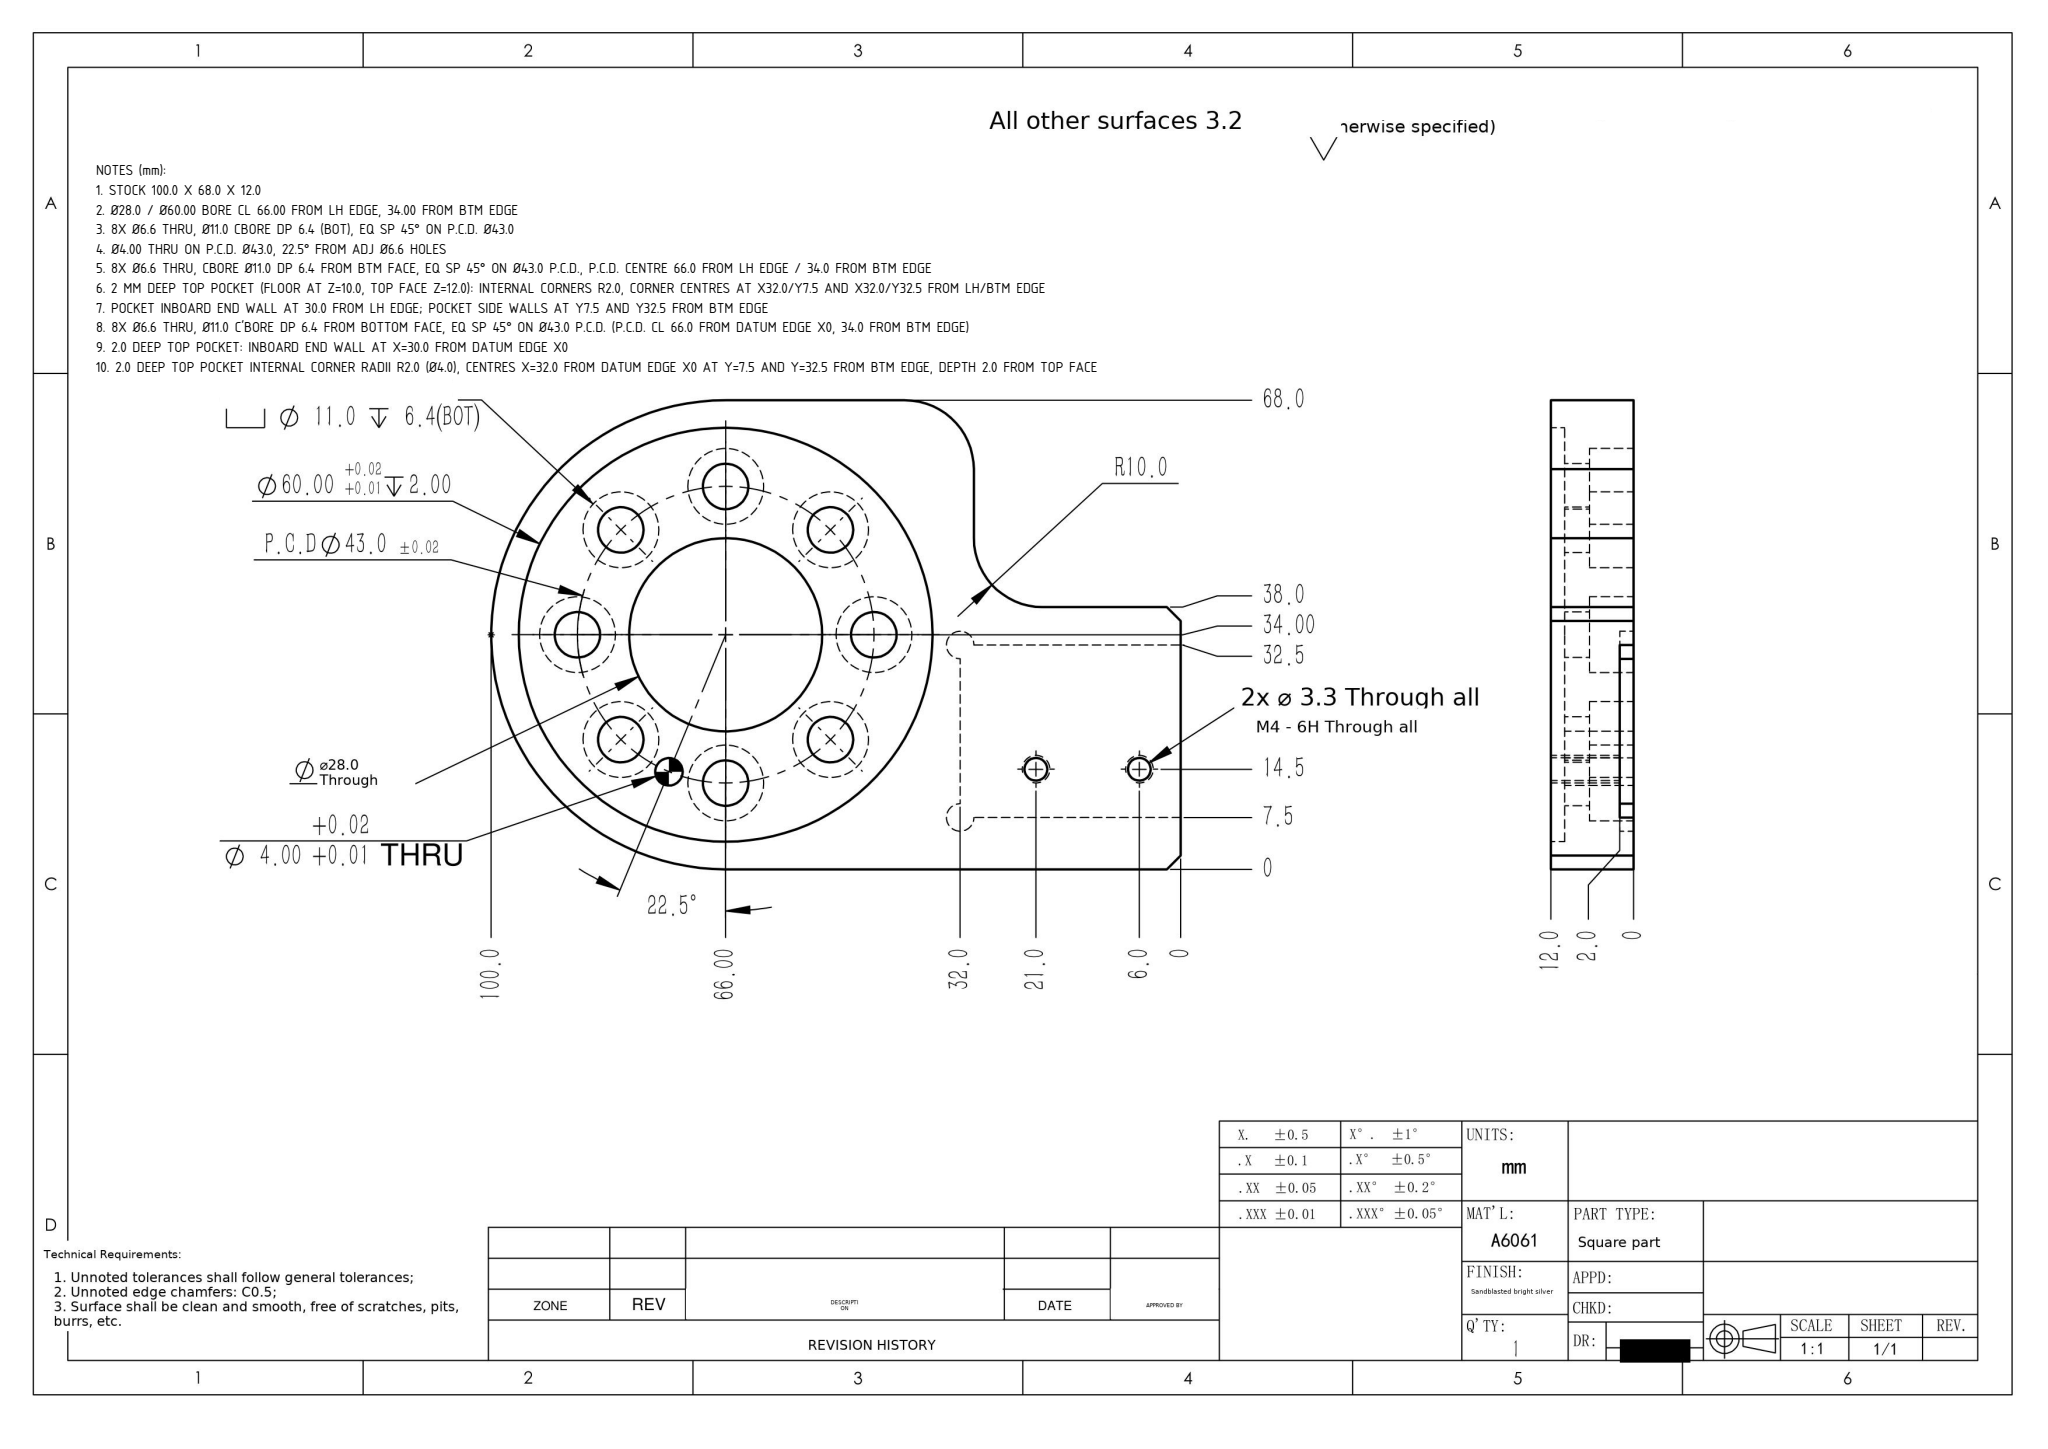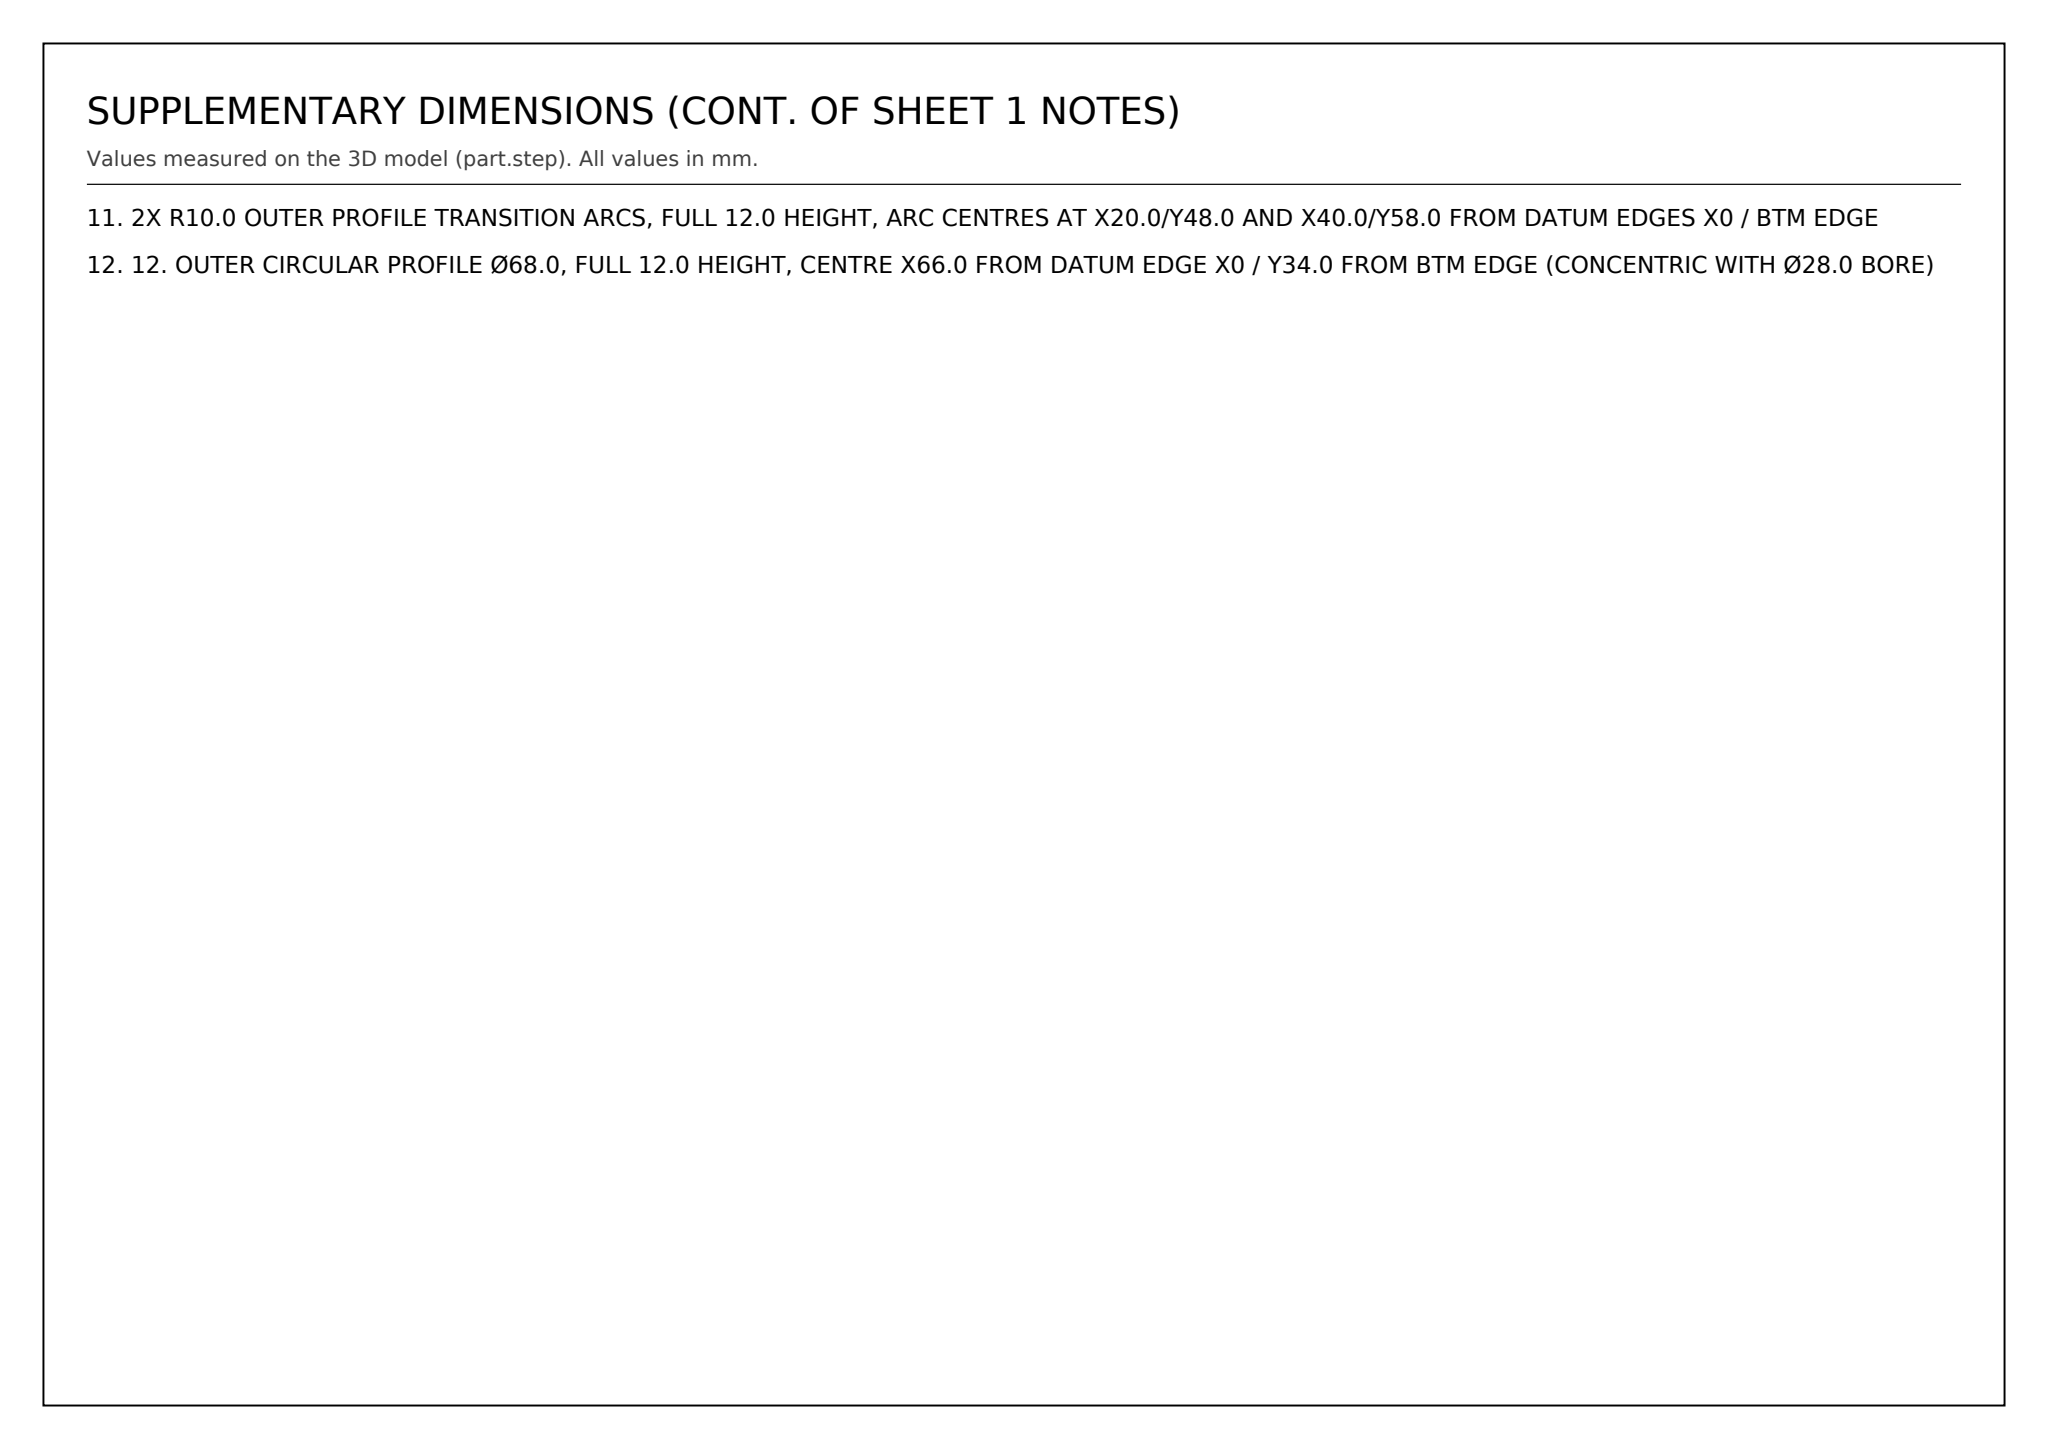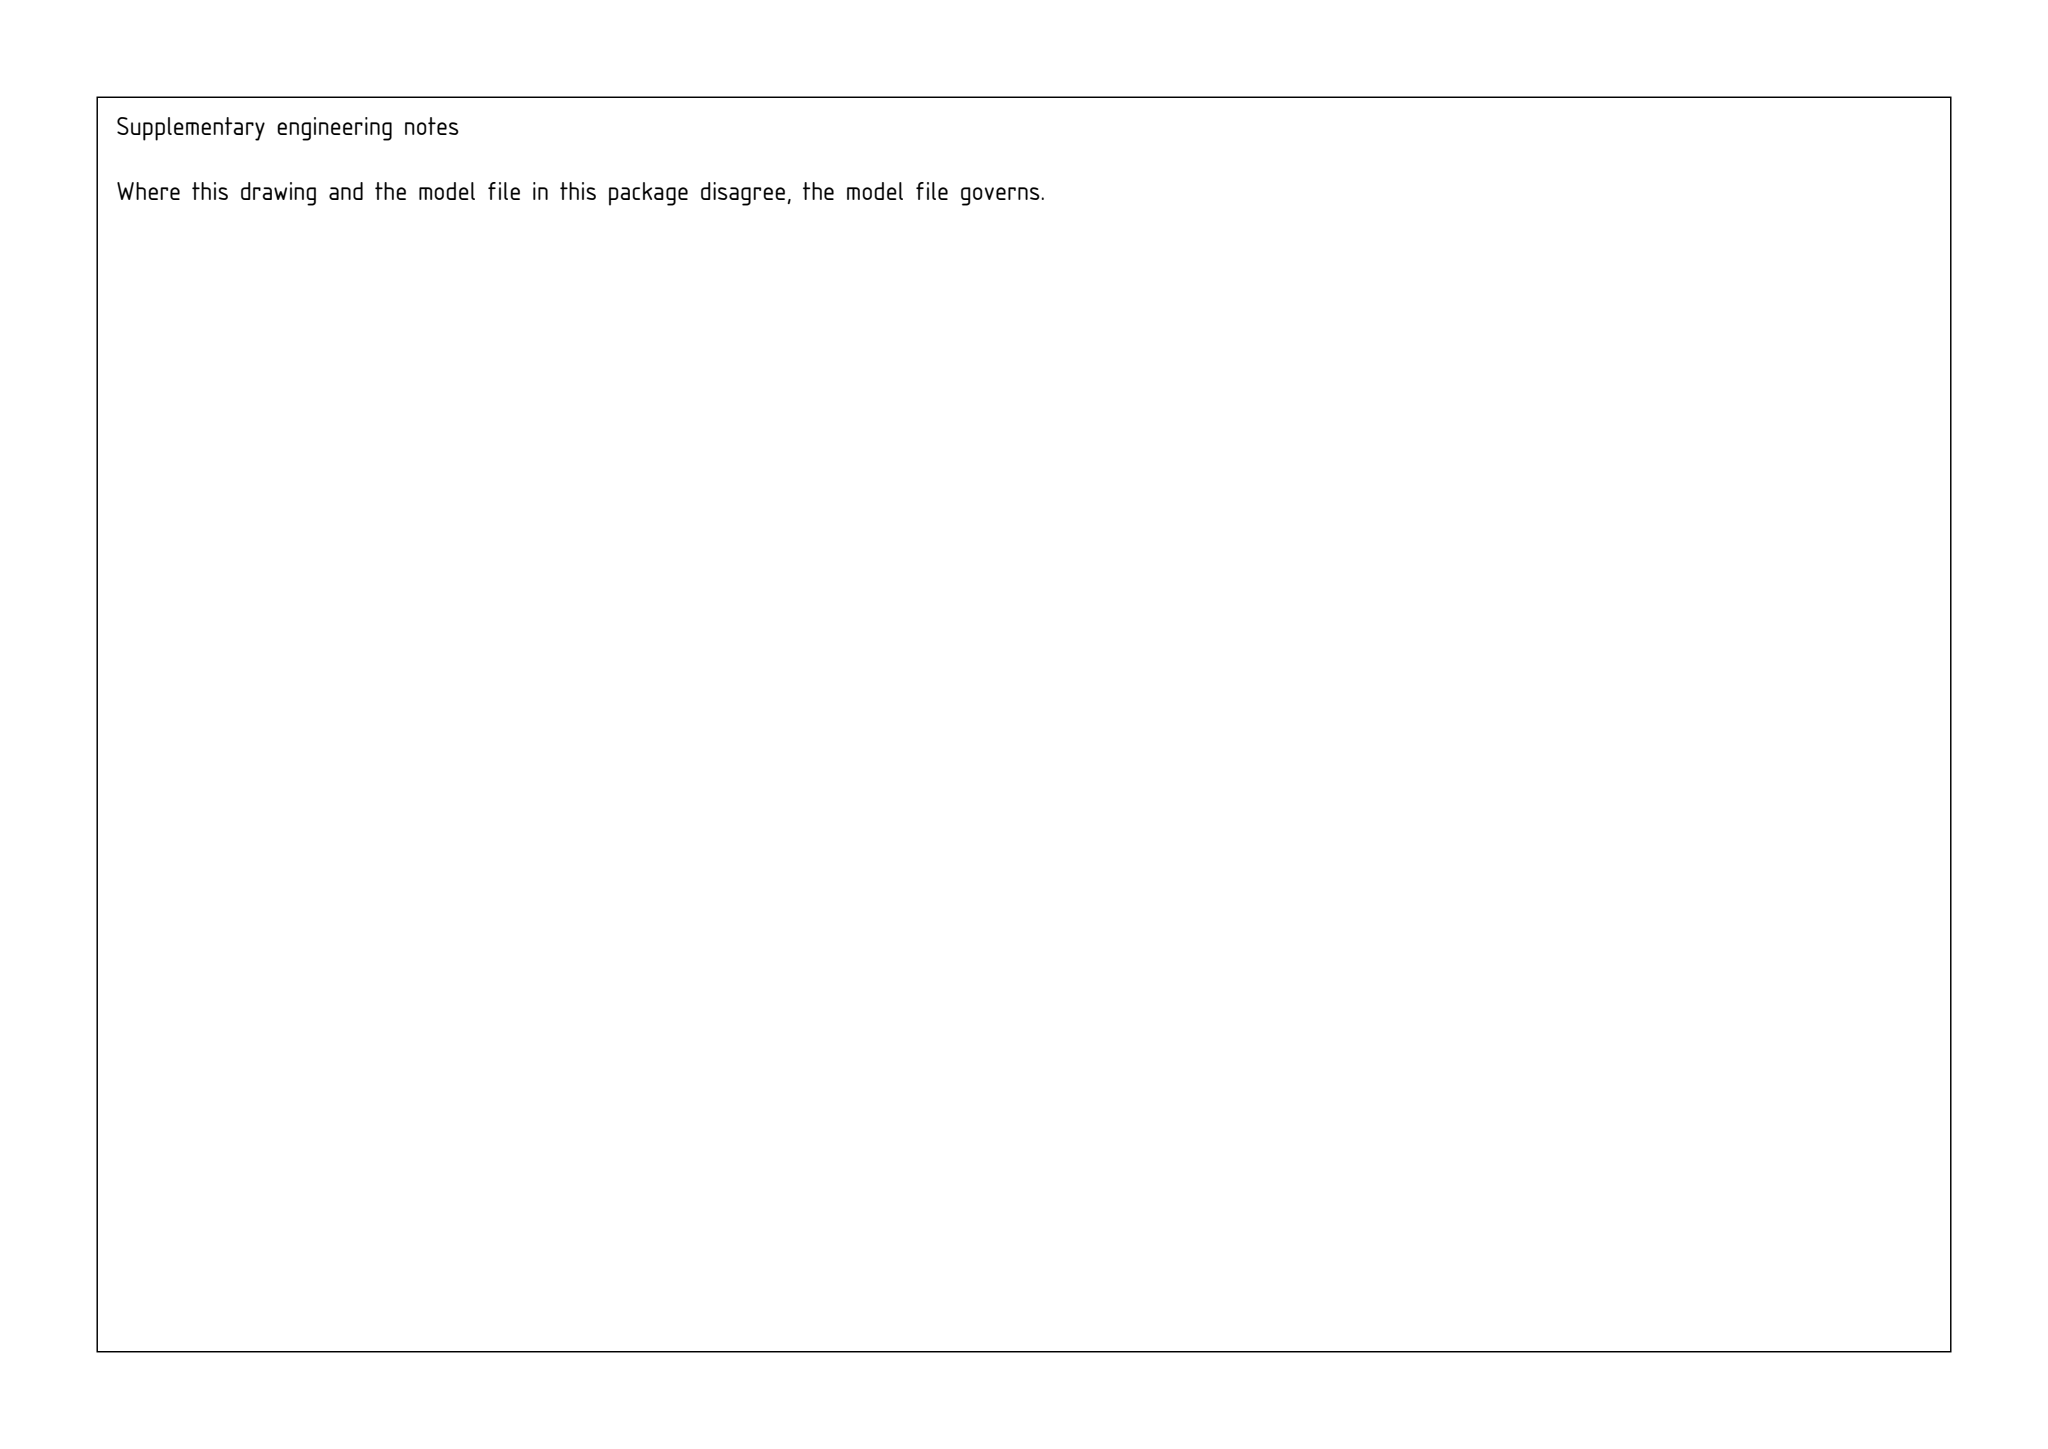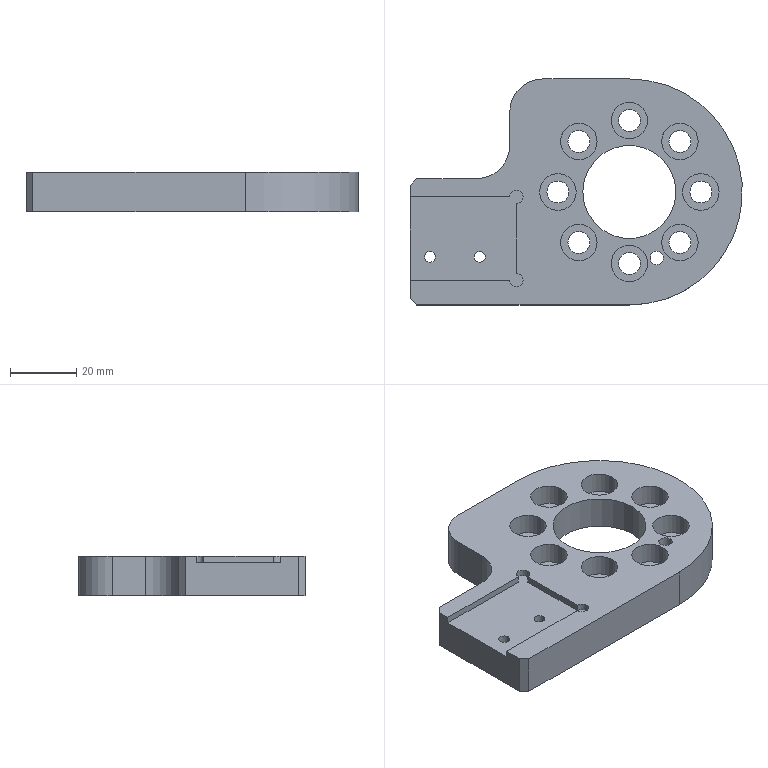Part | SolidWorks | mm | 1 solid | 71 faces | box 100 x 68 x 12 mm | volume 45200 mm3 | cylinder 49 | plane 22 | commonest cylinder face diameters 11 x16 6.6 x16 4 x6 3.3 x4 60 x2 28 x2 20 x2 68 x1
Drawing notes:
STOCK 100.0 X 68.0 X 12.0 | from the solid: bbox_xyz 100.0 x 68.0 x 12.0
Ø28.0 / Ø60.00 BORE CL 66.00 FROM LH EDGE, 34.00 FROM BTM EDGE | from the solid: Ø28.0, Ø60.0 and Ø68.0 cylinders all at pos (66.0, 34.0); datum planes x=0, y=0
8X Ø6.6 THRU, Ø11.0 CBORE DP 6.4 (BOT), EQ SP 45° ON P.C.D. Ø43.0 | from the solid: Eight Ø6.6/Ø11.0 pairs at (44.5,34),(50.8,18.8),(50.8,49.2),(66,12.5),(66,55.5),(81.2,18.8),(81.2,49.2),(87.5,34) - all R21.5 from CL (66,34), 45° spacing
Ø4.00 THRU ON P.C.D. Ø43.0, 22.5° FROM ADJ Ø6.6 HOLES | from the solid: Ø4.0 thru hole at (74.23,14.14): R21.5 from bore CL (66,34), angle -67.5° = 22.5° from holes at -45° and -90°
8X Ø6.6 THRU, CBORE Ø11.0 DP 6.4 FROM BTM FACE, EQ SP 45° ON Ø43.0 P.C.D., P.C.D. CENTRE 66.0 FROM LH EDGE / 34.0 FROM BTM EDGE | from the solid: cylinders dia 6.6 (8 positions, len 3.6) and dia 11.0 (same 8 positions, len 6.4) about centre (66.0, 34.0)
2 MM DEEP TOP POCKET (FLOOR AT Z=10.0, TOP FACE Z=12.0): INTERNAL CORNERS R2.0, CORNER CENTRES AT X32.0/Y7.5 AND X32.0/Y32.5 FROM LH/BTM EDGE | from the solid: cylinders dia 4.0, axis z, pos (32.0,7.5) and (32.0,32.5), length 2.0; planes z=10.0 and z=12.0
POCKET INBOARD END WALL AT 30.0 FROM LH EDGE; POCKET SIDE WALLS AT Y7.5 AND Y32.5 FROM BTM EDGE | from the solid: axis_planes x=30.0, x=32.0, y=7.5, y=32.5
8X Ø6.6 THRU, Ø11.0 C'BORE DP 6.4 FROM BOTTOM FACE, EQ SP 45° ON Ø43.0 P.C.D. (P.C.D. CL 66.0 FROM DATUM EDGE X0, 34.0 FROM BTM EDGE) | from the solid: eight Ø6.6 z-cylinders (44.5,34.0 / 50.8,18.8 / 50.8,49.2 / 66.0,12.5 / 66.0,55.5 / 81.2,18.8 / 81.2,49.2 / 87.5,34.0) each L3.6 with matching eight Ø11.0 cbores L6.4
2.0 DEEP TOP POCKET: INBOARD END WALL AT X=30.0 FROM DATUM EDGE X0 | from the solid: axis_plane normal x, offset 30.0 (with planes y7.5 / y32.5 / z10.0)
2.0 DEEP TOP POCKET INTERNAL CORNER RADII R2.0 (Ø4.0), CENTRES X=32.0 FROM DATUM EDGE X0 AT Y=7.5 AND Y=32.5 FROM BTM EDGE, DEPTH 2.0 FROM TOP FACE | from the solid: cylinders [4.0, z, (32.0,7.5), L2.0] and [4.0, z, (32.0,32.5), L2.0]
2X R10.0 OUTER PROFILE TRANSITION ARCS, FULL 12.0 HEIGHT, ARC CENTRES AT X20.0/Y48.0 AND X40.0/Y58.0 FROM DATUM EDGES X0 / BTM EDGE | from the solid: cylinders [20.0, z, (20.0,48.0), L12.0] and [20.0, z, (40.0,58.0), L12.0]
12. OUTER CIRCULAR PROFILE Ø68.0, FULL 12.0 HEIGHT, CENTRE X66.0 FROM DATUM EDGE X0 / Y34.0 FROM BTM EDGE (CONCENTRIC WITH Ø28.0 BORE) | from the solid: cylinders: [68.0,"z",[66.0,34.0],12.0] outer profile cylinder; bbox_xyz 100.0 x 68.0 x 12.0
build123d program:
from build123d import *

# Parameters (mm, degrees)
BOSS_EXTRUDE1_DEPTH                             = 12
SKETCH2_W                                       = 30
SKETCH2_H                                       = 30
CUT_EXTRUDE1_DEPTH                              = 76.206
SKETCH3_W                                       = 32
SKETCH3_H                                       = 25
CUT_EXTRUDE2_DEPTH                              = 2
SKETCH4_R                                       = 2
CUT_EXTRUDE3_DEPTH                              = 2
SKETCH5_R                                       = 14
CUT_EXTRUDE4_DEPTH                              = 76.206
SKETCH7_R                                       = 30
CUT_EXTRUDE5_DEPTH                              = 2
M6_HEX_SOCKET_HEAD_CAP_SCREW_CBORE1_D           = 6.6
M6_HEX_SOCKET_HEAD_CAP_SCREW_CBORE1_CBORE_D     = 11
M6_HEX_SOCKET_HEAD_CAP_SCREW_CBORE1_CBORE_DEPTH = 6.4
SIZE_MM_DOWEL_PIN_HOLE1_D                       = 4
M4_TAPPED_HOLE1_D                               = 3.3
FILLET1_R                                       = 10
CHAMFER1_SIZE                                   = 2


with BuildPart() as part:
    # Sketch1 → Boss-Extrude1 (new body)
    with BuildSketch(Plane.XY):
        with BuildLine():
            Line((0, 34), (-66, 34))
            Line((-66, 34), (-66, -34))
            Line((-66, -34), (0, -34))
            ThreePointArc((0, -34), (34, 0), (0, 34))
        make_face()
    extrude(amount=BOSS_EXTRUDE1_DEPTH)

    # Sketch2 → Cut-Extrude1 (cut, through all)
    with BuildSketch(Plane.XY.offset(12)):
        with Locations((-51, 19)):
            Rectangle(SKETCH2_W, SKETCH2_H)
    extrude(amount=-CUT_EXTRUDE1_DEPTH, mode=Mode.SUBTRACT)

    # Sketch3 → Cut-Extrude2 (cut)
    with BuildSketch(Plane.XY.offset(12)):
        with Locations((-50, -14)):
            Rectangle(SKETCH3_W, SKETCH3_H)
    extrude(amount=-CUT_EXTRUDE2_DEPTH, mode=Mode.SUBTRACT)

    # Sketch4 → Cut-Extrude3 (cut)
    with BuildSketch(Plane.XY.offset(12)):
        with Locations((-34, -1.5)):
            Circle(SKETCH4_R)
        with Locations((-34, -26.5)):
            Circle(SKETCH4_R)
    extrude(amount=-CUT_EXTRUDE3_DEPTH, mode=Mode.SUBTRACT)

    # Sketch5 → Cut-Extrude4 (cut, through all)
    with BuildSketch(Plane.XY.offset(12)):
        Circle(SKETCH5_R)
    extrude(amount=-CUT_EXTRUDE4_DEPTH, mode=Mode.SUBTRACT)

    # Sketch7 → Cut-Extrude5 (cut)
    with BuildSketch(Plane(origin=(0, 0, 0), x_dir=(-1, 0, 0), z_dir=(0, 0, -1))):
        Circle(SKETCH7_R)
    extrude(amount=-CUT_EXTRUDE5_DEPTH, mode=Mode.SUBTRACT)

    # M6 Hex Socket Head Cap Screw CBORE1 (through all)
    with Locations(Plane.XY.offset(12)):
        with Locations((0, 21.5), (15.203, 15.203), (21.5, 0), (15.203, -15.203), (0, -21.5), (-15.203, -15.203), (-21.5, 0), (-15.203, 15.203), (0, 0)):
            CounterBoreHole(M6_HEX_SOCKET_HEAD_CAP_SCREW_CBORE1_D / 2, M6_HEX_SOCKET_HEAD_CAP_SCREW_CBORE1_CBORE_D / 2, M6_HEX_SOCKET_HEAD_CAP_SCREW_CBORE1_CBORE_DEPTH)

    # Size mm Dowel Pin Hole1 (through all)
    with Locations(Plane.XY.offset(12)):
        with Locations((8.228, -19.863)):
            Hole(SIZE_MM_DOWEL_PIN_HOLE1_D / 2)

    # M4 Tapped Hole1 (through all)
    with Locations(Plane(origin=(0, 0, 0), x_dir=(-1, 0, 0), z_dir=(0, 0, -1))):
        with Locations((45, -19.5), (60, -19.5)):
            Hole(M4_TAPPED_HOLE1_D / 2)

    # Fillet1
    fillet1_edges = [part.edges().sort_by_distance(p)[0] for p in [
        (-36, 34, 6),
        (-36, 4, 6),
    ]]
    fillet(fillet1_edges, radius=FILLET1_R)

    # Chamfer1
    chamfer1_edges = [part.edges().sort_by_distance(p)[0] for p in [
        (-66, 4, 6),
        (-66, -34, 6),
    ]]
    chamfer(chamfer1_edges, length=CHAMFER1_SIZE)


solid = part.part